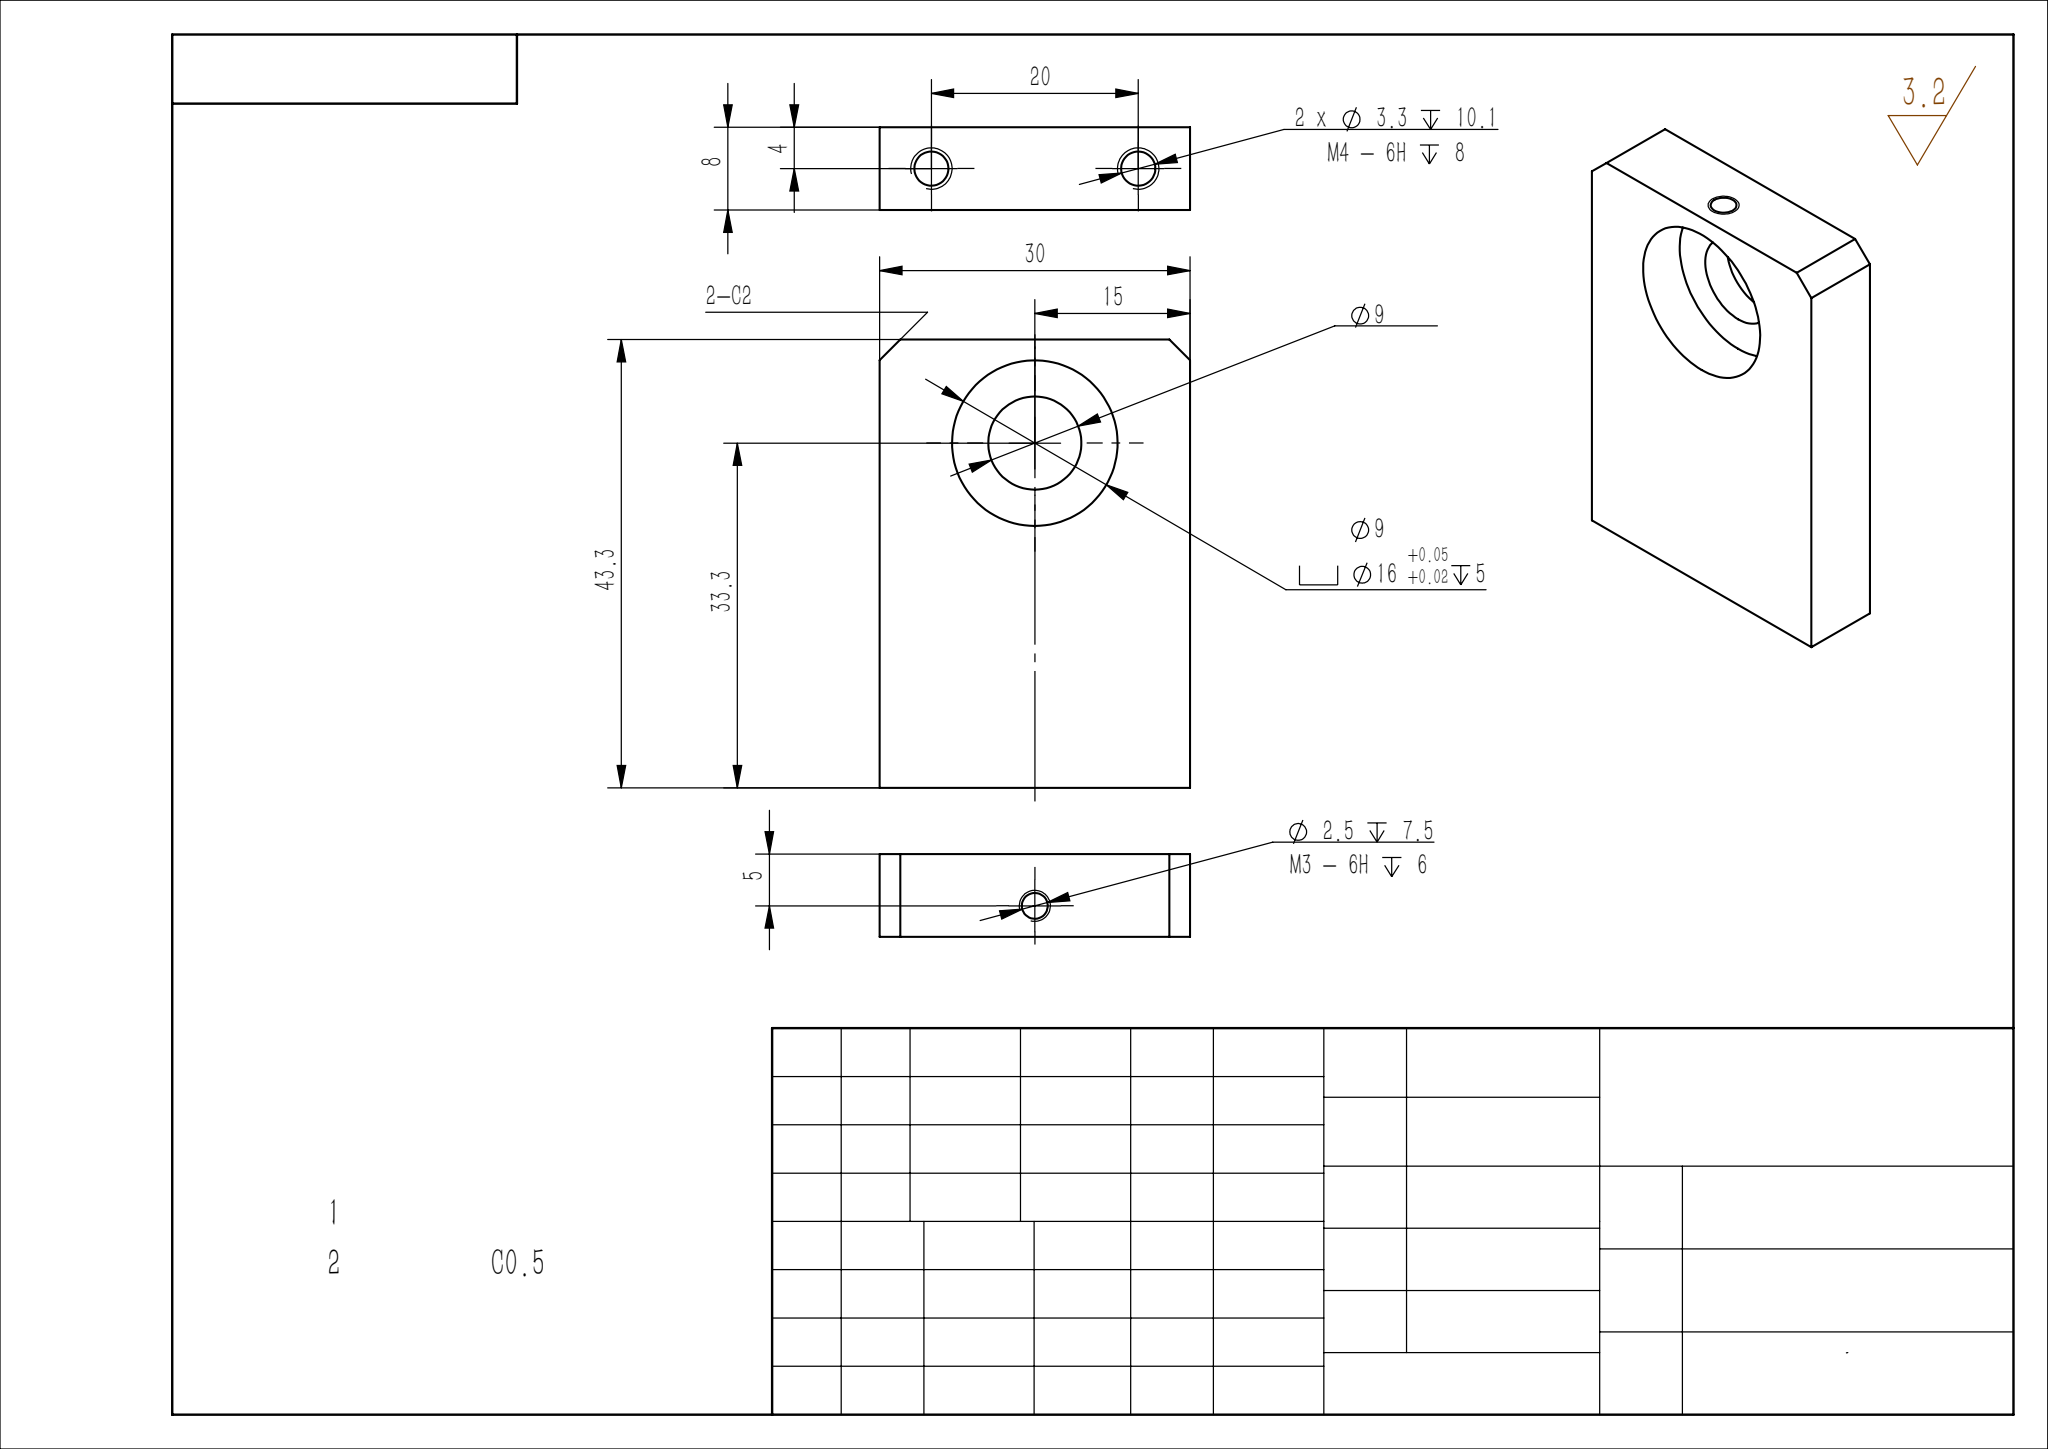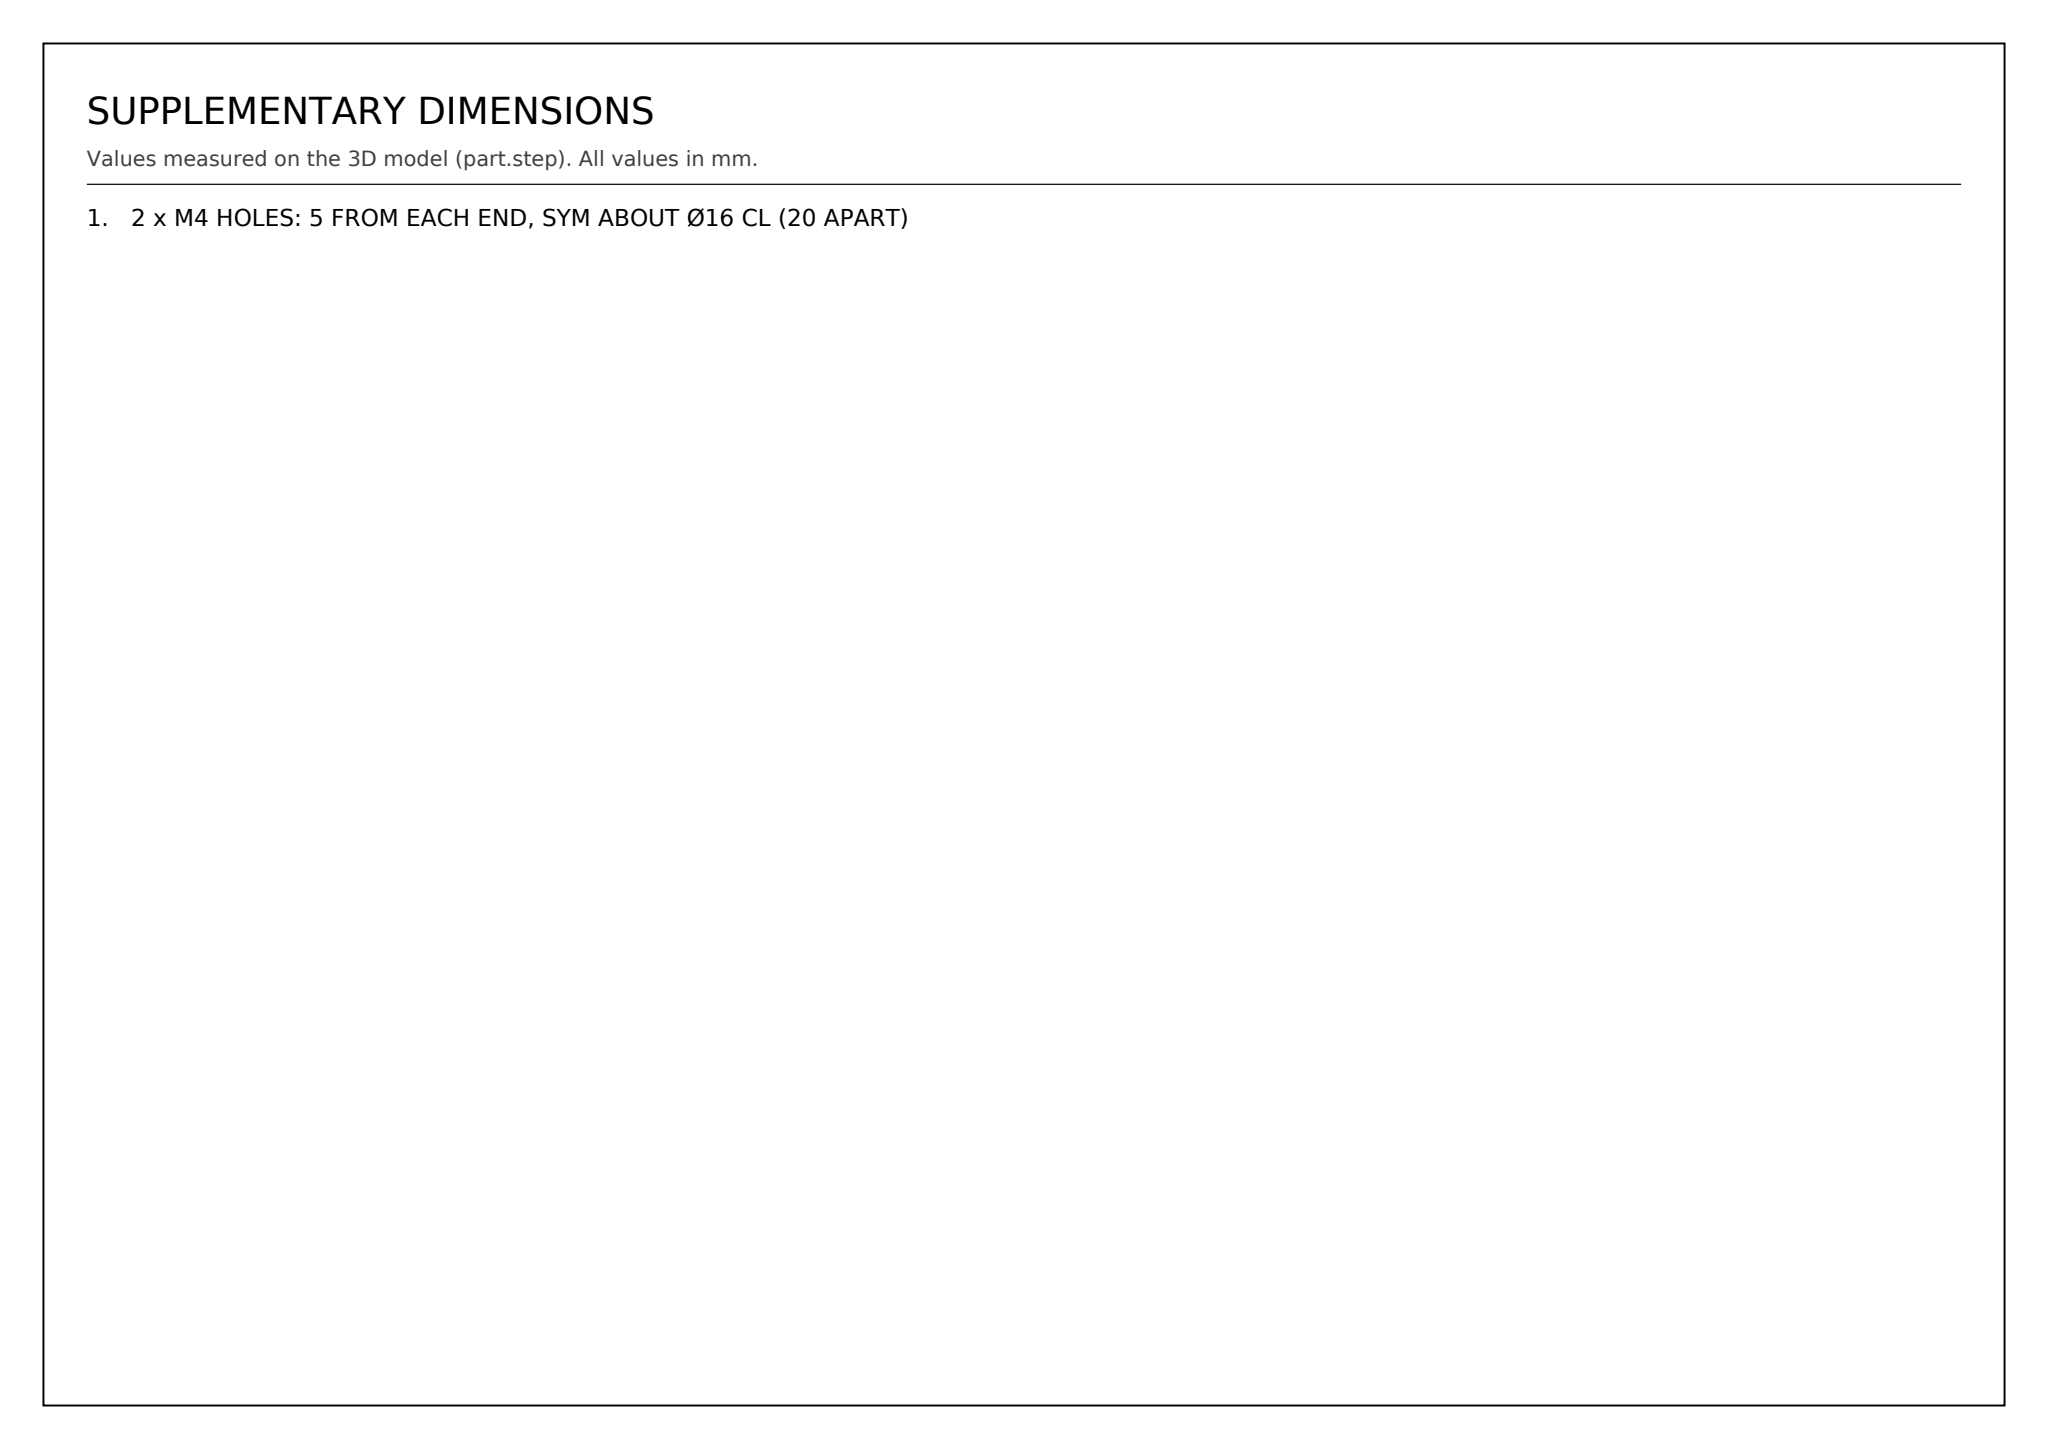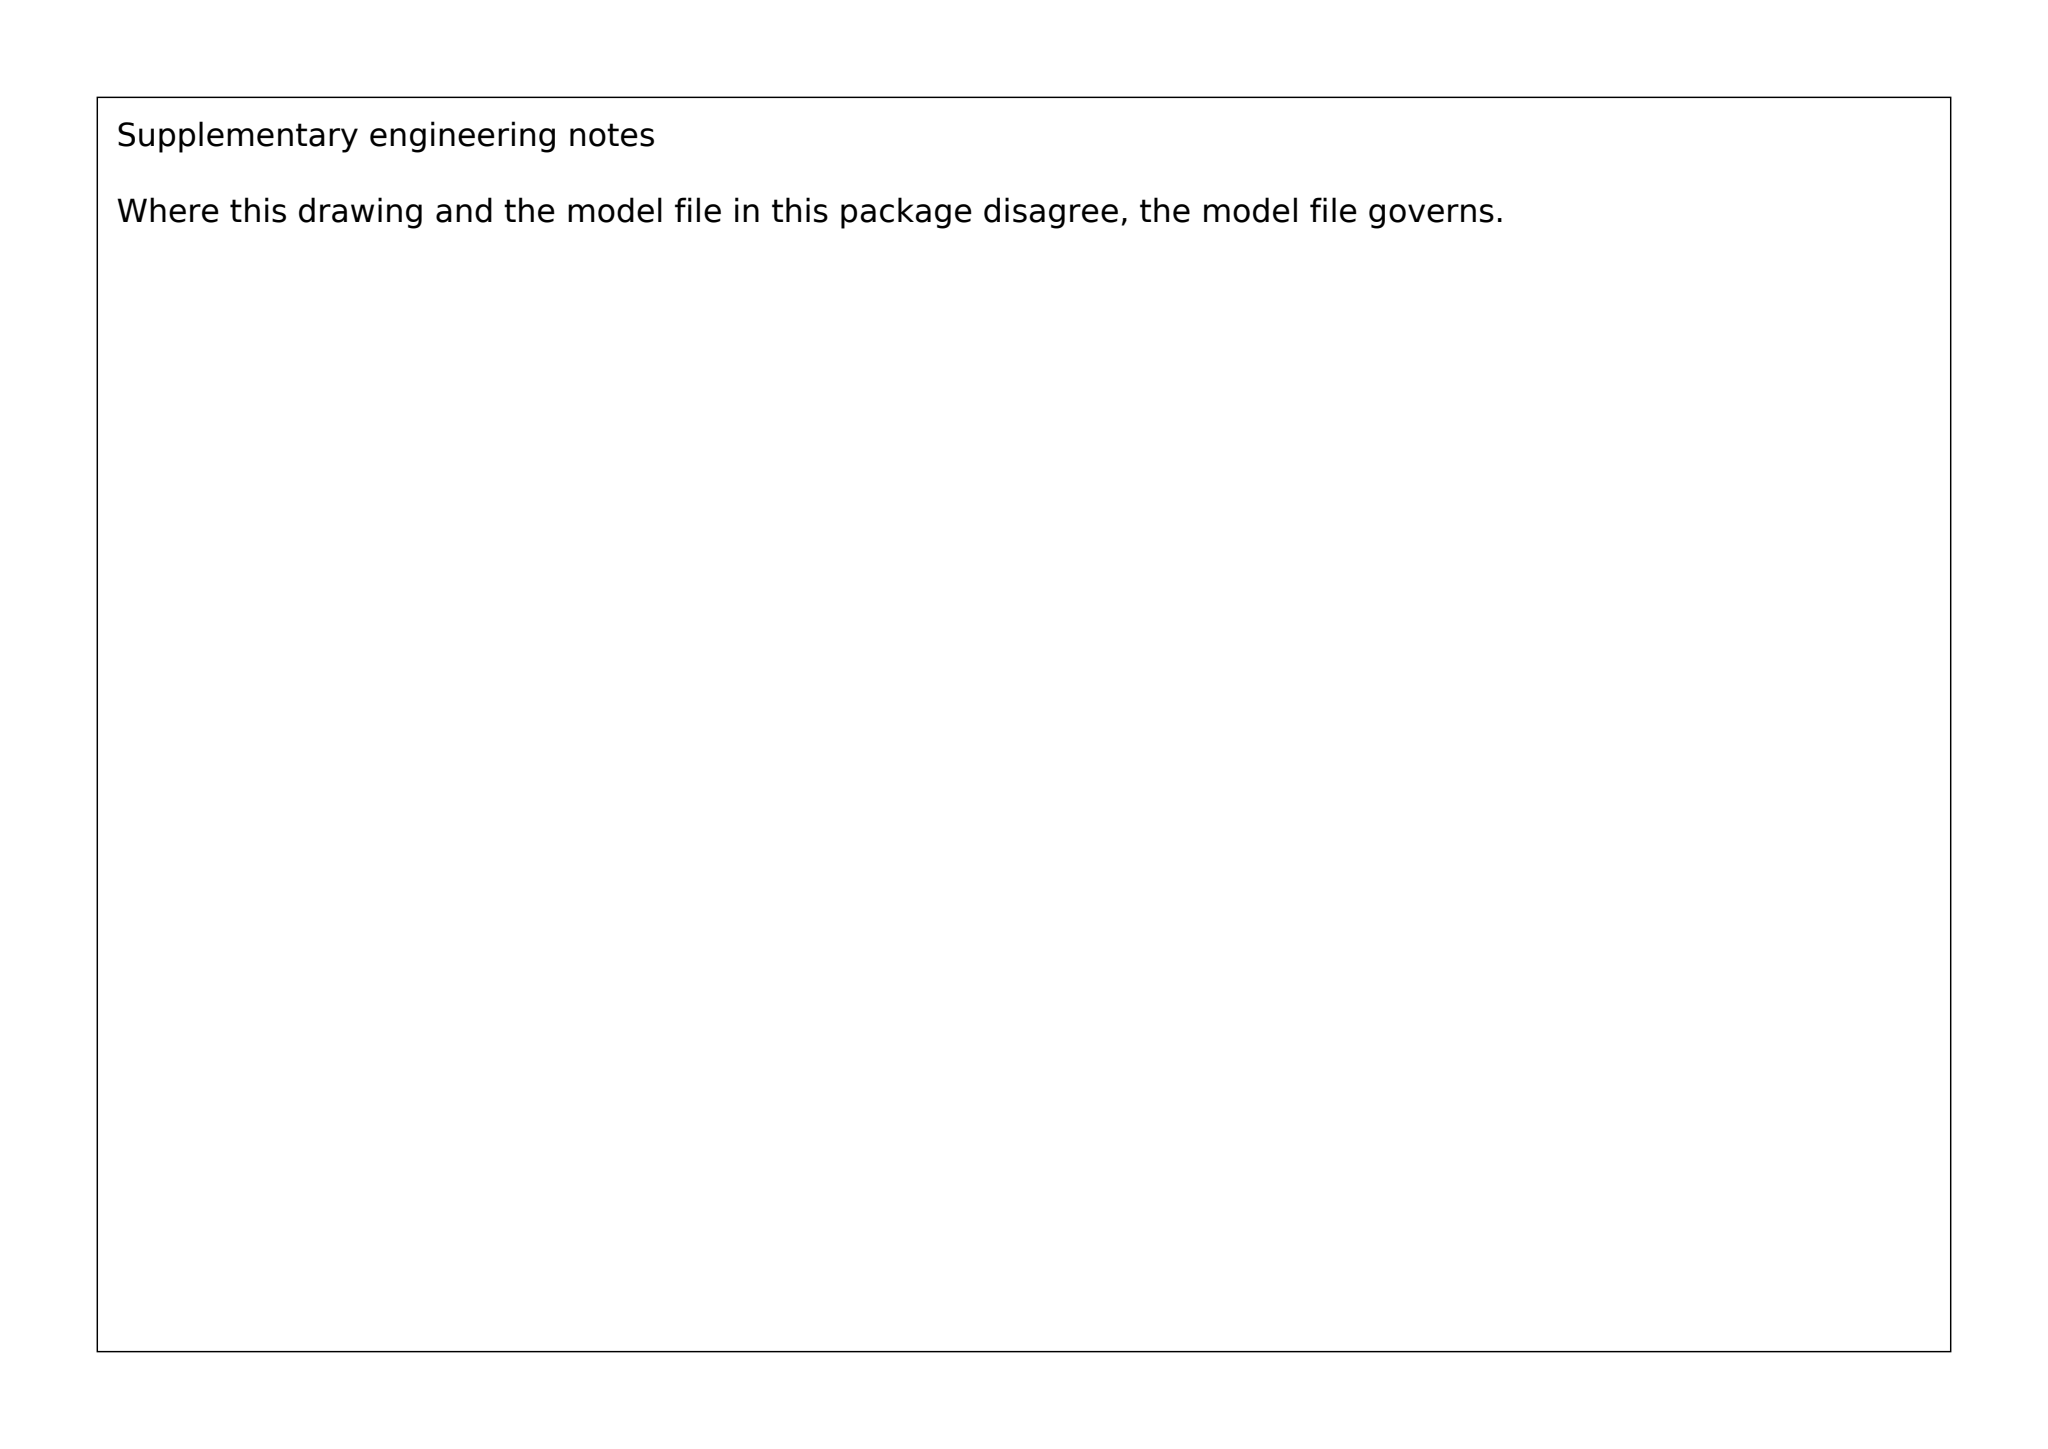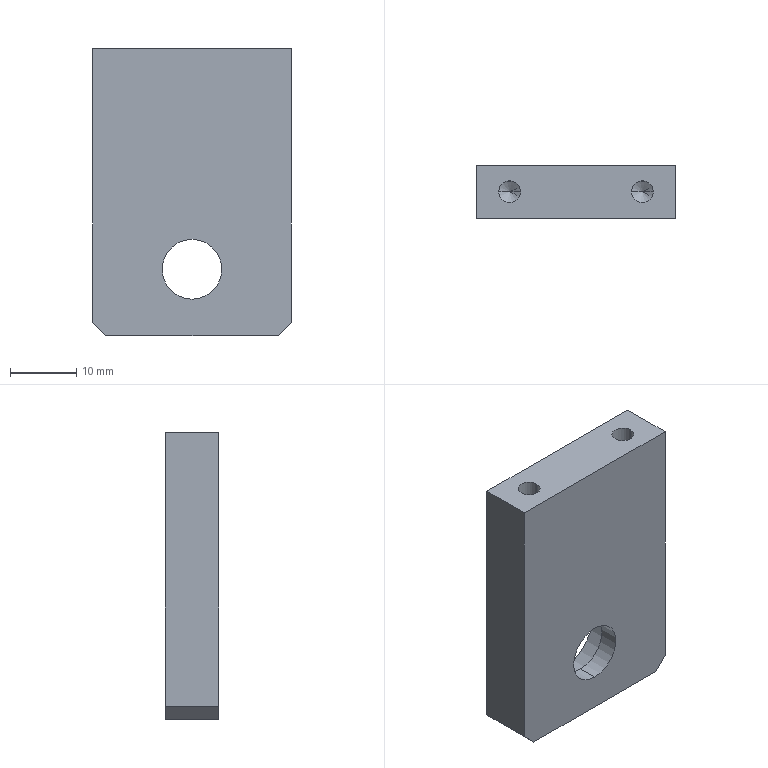Part | SolidWorks | mm | 1 solid | 23 faces | box 30 x 8 x 43.3 mm | volume 8975 mm3 | cylinder 10 | plane 9 | cone 4 | commonest cylinder face diameters 3.3 x4 2.5 x2 9 x2 16 x2
Drawing notes:
2 x M4 HOLES: 5 FROM EACH END, SYM ABOUT Ø16 CL (20 APART) | from the solid: Ø3.3 cyl axes at x=5.0 and x=25.0, bbox X=30.0; Ø16 bore axis at x=15.0
build123d program:
from build123d import *

# Parameters (mm, degrees)
SKETCH1_W             = 30
SKETCH1_H             = 43.3
BOSS_EXTRUDE1_DEPTH   = 8
SKETCH2_R             = 8
CUT_EXTRUDE1_DEPTH    = 5
SKETCH3_R             = 4.5
CUT_EXTRUDE2_DEPTH    = 27.809
CHAMFER1_SIZE         = 2
M4_TAPPED_HOLE1_D     = 3.3
M4_TAPPED_HOLE1_DEPTH = 10.1
M4_TAPPED_HOLE1_TIP   = 0.9914
M3_TAPPED_HOLE1_D     = 2.5
M3_TAPPED_HOLE1_DEPTH = 7.5
M3_TAPPED_HOLE1_TIP   = 0.7511


with BuildPart() as part:
    # Sketch1 → Boss-Extrude1 (new body)
    with BuildSketch(Plane(origin=(0, 0, 0), x_dir=(1, 0, 0), z_dir=(0, 1, 0))):
        Rectangle(SKETCH1_W, SKETCH1_H)
    extrude(amount=BOSS_EXTRUDE1_DEPTH)

    # Sketch2 → Cut-Extrude1 (cut)
    with BuildSketch(Plane(origin=(0, 8, 0), x_dir=(1, 0, 0), z_dir=(0, 1, 0))):
        with Locations(Location((0, 11.65, 0), (0, 0, 270))):
            Circle(SKETCH2_R)
    extrude(amount=-CUT_EXTRUDE1_DEPTH, mode=Mode.SUBTRACT)

    # Sketch3 → Cut-Extrude2 (cut, through all)
    with BuildSketch(Plane(origin=(0, 3, 0), x_dir=(1, 0, 0), z_dir=(0, 1, 0))):
        with Locations(Location((0, 11.65, 0), (0, 0, 270))):
            Circle(SKETCH3_R)
    extrude(amount=-CUT_EXTRUDE2_DEPTH, mode=Mode.SUBTRACT)

    # Chamfer1
    chamfer1_edges = [part.edges().sort_by_distance(p)[0] for p in [
        (-15, 4, -21.65),
        (15, 4, -21.65),
    ]]
    chamfer(chamfer1_edges, length=CHAMFER1_SIZE)

    # M4 Tapped Hole1
    with Locations(Plane.XY.offset(21.65)):
        with Locations((-10, 4), (10, 4)):
            Hole(M4_TAPPED_HOLE1_D / 2, depth=M4_TAPPED_HOLE1_DEPTH)
            with Locations((0, 0, -(M4_TAPPED_HOLE1_DEPTH + M4_TAPPED_HOLE1_TIP / 2))):  # 118° drill point
                Cone(0, M4_TAPPED_HOLE1_D / 2, M4_TAPPED_HOLE1_TIP, mode=Mode.SUBTRACT)

    # M3 Tapped Hole1
    with Locations(Plane(origin=(0, 0, -21.65), x_dir=(-1, 0, 0), z_dir=(0, 0, -1))):
        with Locations((0, 5)):
            Hole(M3_TAPPED_HOLE1_D / 2, depth=M3_TAPPED_HOLE1_DEPTH)
            with Locations((0, 0, -(M3_TAPPED_HOLE1_DEPTH + M3_TAPPED_HOLE1_TIP / 2))):  # 118° drill point
                Cone(0, M3_TAPPED_HOLE1_D / 2, M3_TAPPED_HOLE1_TIP, mode=Mode.SUBTRACT)


solid = part.part